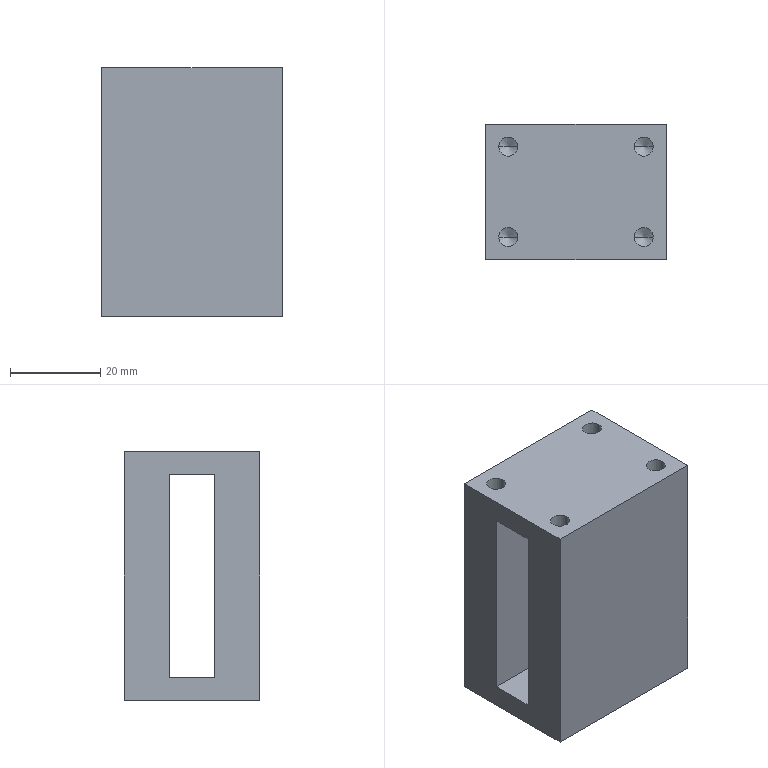Component | SolidWorks | 01-14MarkingMachineMountingSeatPlate-1 | 1 solid | 28 faces | box 40 x 30 x 55 mm | volume 46926 mm3 | cylinder 10 | plane 10 | cone 8 | commonest cylinder face diameters 4.2 x8 6.8 x2 | material A3 Steel
build123d program:
from build123d import *

# Parameters (mm, degrees)
SKETCH1_W             = 55
SKETCH1_H             = 30
SKETCH1_W_2           = 45
SKETCH1_H_2           = 10
BOSS_EXTRUDE1_DEPTH   = 20
M8_TAPPED_HOLE1_D     = 6.8
M8_TAPPED_HOLE1_DEPTH = 10
M5_TAPPED_HOLE1_D     = 4.2
M5_TAPPED_HOLE1_DEPTH = 12.4
M5_TAPPED_HOLE1_TIP   = 1.262


with BuildPart() as part:
    # Sketch1 → Boss-Extrude1 (new, symmetric)
    with BuildSketch(Plane.XY):
        Rectangle(SKETCH1_W, SKETCH1_H)
        Rectangle(SKETCH1_W_2, SKETCH1_H_2, mode=Mode.SUBTRACT)
    extrude(amount=BOSS_EXTRUDE1_DEPTH, both=True)

    # M8 Tapped Hole1
    with Locations(Plane.ZX.offset(15)):
        with Locations((0, 0)):
            Hole(M8_TAPPED_HOLE1_D / 2, depth=M8_TAPPED_HOLE1_DEPTH)

    # M5 Tapped Hole1
    with Locations(Plane(origin=(-27.5, 10, -15), x_dir=(0, 0, -1), z_dir=(-1, 0, 0))):
        with Locations((0, 0), (0, 20), (-30, 0), (-30, 20)):
            Hole(M5_TAPPED_HOLE1_D / 2, depth=M5_TAPPED_HOLE1_DEPTH)
            with Locations((0, 0, -(M5_TAPPED_HOLE1_DEPTH + M5_TAPPED_HOLE1_TIP / 2))):  # 118° drill point
                Cone(0, M5_TAPPED_HOLE1_D / 2, M5_TAPPED_HOLE1_TIP, mode=Mode.SUBTRACT)


solid = part.part

# Placed as in the assembly
solid = solid.moved(Location((-179.532, 2.41, -167.5), (0, 90, 0)))
STEP:
#1=CARTESIAN_POINT('',(-7.741,0.4886,-6.));
#2=VERTEX_POINT('',#1);
#3=CARTESIAN_POINT('',(-7.576,0.4886,-6.));
#4=VERTEX_POINT('',#3);
#5=CARTESIAN_POINT('',(-7.659,0.4886,-6.));
#6=DIRECTION('',(0.,-0.,1.));
#7=DIRECTION('',(1.,0.,0.));
#8=AXIS2_PLACEMENT_3D('',#5,#6,#7);
#9=CIRCLE('',#8,0.08268);
#10=EDGE_CURVE('',#2,#4,#9,.T.);
#11=ORIENTED_EDGE('',*,*,#10,.F.);
#12=CARTESIAN_POINT('',(-7.741,0.4886,-5.512));
#13=VERTEX_POINT('',#12);
#14=CARTESIAN_POINT('',(-7.741,0.4886,-5.512));
#15=DIRECTION('',(0.,-0.,1.));
#16=VECTOR('',#15,39.37);
#17=LINE('',#14,#16);
#18=EDGE_CURVE('',#2,#13,#17,.T.);
#19=ORIENTED_EDGE('',*,*,#18,.T.);
#20=CARTESIAN_POINT('',(-7.576,0.4886,-5.512));
#21=VERTEX_POINT('',#20);
#22=CARTESIAN_POINT('',(-7.659,0.4886,-5.512));
#23=DIRECTION('',(0.,-0.,1.));
#24=DIRECTION('',(1.,0.,0.));
#25=AXIS2_PLACEMENT_3D('',#22,#23,#24);
#26=CIRCLE('',#25,0.08268);
#27=EDGE_CURVE('',#13,#21,#26,.T.);
#28=ORIENTED_EDGE('',*,*,#27,.T.);
#29=CARTESIAN_POINT('',(-7.576,0.4886,-5.512));
#30=DIRECTION('',(0.,-0.,1.));
#31=VECTOR('',#30,39.37);
#32=LINE('',#29,#31);
#33=EDGE_CURVE('',#4,#21,#32,.T.);
#34=ORIENTED_EDGE('',*,*,#33,.F.);
#35=EDGE_LOOP('',(#11,#19,#28,#34));
#36=FACE_OUTER_BOUND('',#35,.T.);
#37=CARTESIAN_POINT('',(-7.659,0.4886,-5.512));
#38=DIRECTION('',(0.,-0.,1.));
#39=DIRECTION('',(1.,0.,0.));
#40=AXIS2_PLACEMENT_3D('',#37,#38,#39);
#41=CYLINDRICAL_SURFACE('',#40,0.08268);
#42=ADVANCED_FACE('',(#36),#41,.F.);
#43=CARTESIAN_POINT('',(-7.659,0.4886,-6.05));
#44=VERTEX_POINT('',#43);
#45=CARTESIAN_POINT('',(-7.576,0.4886,-6.));
#46=DIRECTION('',(0.8572,0.,0.515));
#47=VECTOR('',#46,39.37);
#48=LINE('',#45,#47);
#49=EDGE_CURVE('',#44,#4,#48,.T.);
#50=ORIENTED_EDGE('',*,*,#49,.F.);
#51=CARTESIAN_POINT('',(-7.741,0.4886,-6.));
#52=DIRECTION('',(-0.8572,-0.,0.515));
#53=VECTOR('',#52,39.37);
#54=LINE('',#51,#53);
#55=EDGE_CURVE('',#44,#2,#54,.T.);
#56=ORIENTED_EDGE('',*,*,#55,.T.);
#57=ORIENTED_EDGE('',*,*,#10,.T.);
#58=EDGE_LOOP('',(#50,#56,#57));
#59=FACE_OUTER_BOUND('',#58,.T.);
#60=CARTESIAN_POINT('',(-7.659,0.4886,-6.));
#61=DIRECTION('',(0.,-0.,1.));
#62=DIRECTION('',(1.,0.,0.));
#63=AXIS2_PLACEMENT_3D('',#60,#61,#62);
#64=CONICAL_SURFACE('',#63,0.08268,1.03);
#65=ADVANCED_FACE('',(#59),#64,.F.);
#66=CARTESIAN_POINT('',(-7.741,-0.2988,-6.));
#67=VERTEX_POINT('',#66);
#68=CARTESIAN_POINT('',(-7.576,-0.2988,-6.));
#69=VERTEX_POINT('',#68);
#70=CARTESIAN_POINT('',(-7.659,-0.2988,-6.));
#71=DIRECTION('',(0.,-0.,1.));
#72=DIRECTION('',(1.,0.,0.));
#73=AXIS2_PLACEMENT_3D('',#70,#71,#72);
#74=CIRCLE('',#73,0.08268);
#75=EDGE_CURVE('',#67,#69,#74,.T.);
#76=ORIENTED_EDGE('',*,*,#75,.F.);
#77=CARTESIAN_POINT('',(-7.741,-0.2988,-5.512));
#78=VERTEX_POINT('',#77);
#79=CARTESIAN_POINT('',(-7.741,-0.2988,-5.512));
#80=DIRECTION('',(0.,-0.,1.));
#81=VECTOR('',#80,39.37);
#82=LINE('',#79,#81);
#83=EDGE_CURVE('',#67,#78,#82,.T.);
#84=ORIENTED_EDGE('',*,*,#83,.T.);
#85=CARTESIAN_POINT('',(-7.576,-0.2988,-5.512));
#86=VERTEX_POINT('',#85);
#87=CARTESIAN_POINT('',(-7.659,-0.2988,-5.512));
#88=DIRECTION('',(0.,-0.,1.));
#89=DIRECTION('',(1.,0.,0.));
#90=AXIS2_PLACEMENT_3D('',#87,#88,#89);
#91=CIRCLE('',#90,0.08268);
#92=EDGE_CURVE('',#78,#86,#91,.T.);
#93=ORIENTED_EDGE('',*,*,#92,.T.);
#94=CARTESIAN_POINT('',(-7.576,-0.2988,-5.512));
#95=DIRECTION('',(0.,-0.,1.));
#96=VECTOR('',#95,39.37);
#97=LINE('',#94,#96);
#98=EDGE_CURVE('',#69,#86,#97,.T.);
#99=ORIENTED_EDGE('',*,*,#98,.F.);
#100=EDGE_LOOP('',(#76,#84,#93,#99));
#101=FACE_OUTER_BOUND('',#100,.T.);
#102=CARTESIAN_POINT('',(-7.659,-0.2988,-5.512));
#103=DIRECTION('',(0.,-0.,1.));
#104=DIRECTION('',(1.,0.,0.));
#105=AXIS2_PLACEMENT_3D('',#102,#103,#104);
#106=CYLINDRICAL_SURFACE('',#105,0.08268);
#107=ADVANCED_FACE('',(#101),#106,.F.);
#108=CARTESIAN_POINT('',(-7.659,-0.2988,-6.05));
#109=VERTEX_POINT('',#108);
#110=CARTESIAN_POINT('',(-7.576,-0.2988,-6.));
#111=DIRECTION('',(0.8572,0.,0.515));
#112=VECTOR('',#111,39.37);
#113=LINE('',#110,#112);
#114=EDGE_CURVE('',#109,#69,#113,.T.);
#115=ORIENTED_EDGE('',*,*,#114,.F.);
#116=CARTESIAN_POINT('',(-7.741,-0.2988,-6.));
#117=DIRECTION('',(-0.8572,-0.,0.515));
#118=VECTOR('',#117,39.37);
#119=LINE('',#116,#118);
#120=EDGE_CURVE('',#109,#67,#119,.T.);
#121=ORIENTED_EDGE('',*,*,#120,.T.);
#122=ORIENTED_EDGE('',*,*,#75,.T.);
#123=EDGE_LOOP('',(#115,#121,#122));
#124=FACE_OUTER_BOUND('',#123,.T.);
#125=CARTESIAN_POINT('',(-7.659,-0.2988,-6.));
#126=DIRECTION('',(0.,-0.,1.));
#127=DIRECTION('',(1.,0.,0.));
#128=AXIS2_PLACEMENT_3D('',#125,#126,#127);
#129=CONICAL_SURFACE('',#128,0.08268,1.03);
#130=ADVANCED_FACE('',(#124),#129,.F.);
#131=CARTESIAN_POINT('',(-6.56,0.4886,-6.));
#132=VERTEX_POINT('',#131);
#133=CARTESIAN_POINT('',(-6.395,0.4886,-6.));
#134=VERTEX_POINT('',#133);
#135=CARTESIAN_POINT('',(-6.478,0.4886,-6.));
#136=DIRECTION('',(0.,-0.,1.));
#137=DIRECTION('',(1.,0.,0.));
#138=AXIS2_PLACEMENT_3D('',#135,#136,#137);
#139=CIRCLE('',#138,0.08268);
#140=EDGE_CURVE('',#132,#134,#139,.T.);
#141=ORIENTED_EDGE('',*,*,#140,.F.);
#142=CARTESIAN_POINT('',(-6.56,0.4886,-5.512));
#143=VERTEX_POINT('',#142);
#144=CARTESIAN_POINT('',(-6.56,0.4886,-5.512));
#145=DIRECTION('',(0.,-0.,1.));
#146=VECTOR('',#145,39.37);
#147=LINE('',#144,#146);
#148=EDGE_CURVE('',#132,#143,#147,.T.);
#149=ORIENTED_EDGE('',*,*,#148,.T.);
#150=CARTESIAN_POINT('',(-6.395,0.4886,-5.512));
#151=VERTEX_POINT('',#150);
#152=CARTESIAN_POINT('',(-6.478,0.4886,-5.512));
#153=DIRECTION('',(0.,-0.,1.));
#154=DIRECTION('',(1.,0.,0.));
#155=AXIS2_PLACEMENT_3D('',#152,#153,#154);
#156=CIRCLE('',#155,0.08268);
#157=EDGE_CURVE('',#143,#151,#156,.T.);
#158=ORIENTED_EDGE('',*,*,#157,.T.);
#159=CARTESIAN_POINT('',(-6.395,0.4886,-5.512));
#160=DIRECTION('',(0.,-0.,1.));
#161=VECTOR('',#160,39.37);
#162=LINE('',#159,#161);
#163=EDGE_CURVE('',#134,#151,#162,.T.);
#164=ORIENTED_EDGE('',*,*,#163,.F.);
#165=EDGE_LOOP('',(#141,#149,#158,#164));
#166=FACE_OUTER_BOUND('',#165,.T.);
#167=CARTESIAN_POINT('',(-6.478,0.4886,-5.512));
#168=DIRECTION('',(0.,-0.,1.));
#169=DIRECTION('',(1.,0.,0.));
#170=AXIS2_PLACEMENT_3D('',#167,#168,#169);
#171=CYLINDRICAL_SURFACE('',#170,0.08268);
#172=ADVANCED_FACE('',(#166),#171,.F.);
#173=CARTESIAN_POINT('',(-6.478,0.4886,-6.05));
#174=VERTEX_POINT('',#173);
#175=CARTESIAN_POINT('',(-6.395,0.4886,-6.));
#176=DIRECTION('',(0.8572,0.,0.515));
#177=VECTOR('',#176,39.37);
#178=LINE('',#175,#177);
#179=EDGE_CURVE('',#174,#134,#178,.T.);
#180=ORIENTED_EDGE('',*,*,#179,.F.);
#181=CARTESIAN_POINT('',(-6.56,0.4886,-6.));
#182=DIRECTION('',(-0.8572,-0.,0.515));
#183=VECTOR('',#182,39.37);
#184=LINE('',#181,#183);
#185=EDGE_CURVE('',#174,#132,#184,.T.);
#186=ORIENTED_EDGE('',*,*,#185,.T.);
#187=ORIENTED_EDGE('',*,*,#140,.T.);
#188=EDGE_LOOP('',(#180,#186,#187));
#189=FACE_OUTER_BOUND('',#188,.T.);
#190=CARTESIAN_POINT('',(-6.478,0.4886,-6.));
#191=DIRECTION('',(0.,-0.,1.));
#192=DIRECTION('',(1.,0.,0.));
#193=AXIS2_PLACEMENT_3D('',#190,#191,#192);
#194=CONICAL_SURFACE('',#193,0.08268,1.03);
#195=ADVANCED_FACE('',(#189),#194,.F.);
#196=CARTESIAN_POINT('',(-6.56,-0.2988,-6.));
#197=VERTEX_POINT('',#196);
#198=CARTESIAN_POINT('',(-6.395,-0.2988,-6.));
#199=VERTEX_POINT('',#198);
#200=CARTESIAN_POINT('',(-6.478,-0.2988,-6.));
#201=DIRECTION('',(0.,-0.,1.));
#202=DIRECTION('',(1.,0.,0.));
#203=AXIS2_PLACEMENT_3D('',#200,#201,#202);
#204=CIRCLE('',#203,0.08268);
#205=EDGE_CURVE('',#197,#199,#204,.T.);
#206=ORIENTED_EDGE('',*,*,#205,.F.);
#207=CARTESIAN_POINT('',(-6.56,-0.2988,-5.512));
#208=VERTEX_POINT('',#207);
#209=CARTESIAN_POINT('',(-6.56,-0.2988,-5.512));
#210=DIRECTION('',(0.,-0.,1.));
#211=VECTOR('',#210,39.37);
#212=LINE('',#209,#211);
#213=EDGE_CURVE('',#197,#208,#212,.T.);
#214=ORIENTED_EDGE('',*,*,#213,.T.);
#215=CARTESIAN_POINT('',(-6.395,-0.2988,-5.512));
#216=VERTEX_POINT('',#215);
#217=CARTESIAN_POINT('',(-6.478,-0.2988,-5.512));
#218=DIRECTION('',(0.,-0.,1.));
#219=DIRECTION('',(1.,0.,0.));
#220=AXIS2_PLACEMENT_3D('',#217,#218,#219);
#221=CIRCLE('',#220,0.08268);
#222=EDGE_CURVE('',#208,#216,#221,.T.);
#223=ORIENTED_EDGE('',*,*,#222,.T.);
#224=CARTESIAN_POINT('',(-6.395,-0.2988,-5.512));
#225=DIRECTION('',(0.,-0.,1.));
#226=VECTOR('',#225,39.37);
#227=LINE('',#224,#226);
#228=EDGE_CURVE('',#199,#216,#227,.T.);
#229=ORIENTED_EDGE('',*,*,#228,.F.);
#230=EDGE_LOOP('',(#206,#214,#223,#229));
#231=FACE_OUTER_BOUND('',#230,.T.);
#232=CARTESIAN_POINT('',(-6.478,-0.2988,-5.512));
#233=DIRECTION('',(0.,-0.,1.));
#234=DIRECTION('',(1.,0.,0.));
#235=AXIS2_PLACEMENT_3D('',#232,#233,#234);
#236=CYLINDRICAL_SURFACE('',#235,0.08268);
#237=ADVANCED_FACE('',(#231),#236,.F.);
#238=CARTESIAN_POINT('',(-6.478,-0.2988,-6.05));
#239=VERTEX_POINT('',#238);
#240=CARTESIAN_POINT('',(-6.395,-0.2988,-6.));
#241=DIRECTION('',(0.8572,0.,0.515));
#242=VECTOR('',#241,39.37);
#243=LINE('',#240,#242);
#244=EDGE_CURVE('',#239,#199,#243,.T.);
#245=ORIENTED_EDGE('',*,*,#244,.F.);
#246=CARTESIAN_POINT('',(-6.56,-0.2988,-6.));
#247=DIRECTION('',(-0.8572,-0.,0.515));
#248=VECTOR('',#247,39.37);
#249=LINE('',#246,#248);
#250=EDGE_CURVE('',#239,#197,#249,.T.);
#251=ORIENTED_EDGE('',*,*,#250,.T.);
#252=ORIENTED_EDGE('',*,*,#205,.T.);
#253=EDGE_LOOP('',(#245,#251,#252));
#254=FACE_OUTER_BOUND('',#253,.T.);
#255=CARTESIAN_POINT('',(-6.478,-0.2988,-6.));
#256=DIRECTION('',(0.,-0.,1.));
#257=DIRECTION('',(1.,0.,0.));
#258=AXIS2_PLACEMENT_3D('',#255,#256,#257);
#259=CONICAL_SURFACE('',#258,0.08268,1.03);
#260=ADVANCED_FACE('',(#254),#259,.F.);
#261=CARTESIAN_POINT('',(-6.934,0.2918,-6.594));
#262=VERTEX_POINT('',#261);
#263=CARTESIAN_POINT('',(-7.202,0.2918,-6.594));
#264=VERTEX_POINT('',#263);
#265=CARTESIAN_POINT('',(-7.068,0.2918,-6.594));
#266=DIRECTION('',(0.,-1.,-0.));
#267=DIRECTION('',(-1.,0.,0.));
#268=AXIS2_PLACEMENT_3D('',#265,#266,#267);
#269=CIRCLE('',#268,0.1339);
#270=EDGE_CURVE('',#262,#264,#269,.T.);
#271=ORIENTED_EDGE('',*,*,#270,.T.);
#272=CARTESIAN_POINT('',(-7.202,0.6855,-6.594));
#273=VERTEX_POINT('',#272);
#274=CARTESIAN_POINT('',(-7.202,0.6855,-6.594));
#275=DIRECTION('',(-0.,1.,0.));
#276=VECTOR('',#275,39.37);
#277=LINE('',#274,#276);
#278=EDGE_CURVE('',#264,#273,#277,.T.);
#279=ORIENTED_EDGE('',*,*,#278,.T.);
#280=CARTESIAN_POINT('',(-6.934,0.6855,-6.594));
#281=VERTEX_POINT('',#280);
#282=CARTESIAN_POINT('',(-7.068,0.6855,-6.594));
#283=DIRECTION('',(-0.,1.,0.));
#284=DIRECTION('',(1.,0.,0.));
#285=AXIS2_PLACEMENT_3D('',#282,#283,#284);
#286=CIRCLE('',#285,0.1339);
#287=EDGE_CURVE('',#273,#281,#286,.T.);
#288=ORIENTED_EDGE('',*,*,#287,.T.);
#289=CARTESIAN_POINT('',(-6.934,0.6855,-6.594));
#290=DIRECTION('',(-0.,1.,0.));
#291=VECTOR('',#290,39.37);
#292=LINE('',#289,#291);
#293=EDGE_CURVE('',#262,#281,#292,.T.);
#294=ORIENTED_EDGE('',*,*,#293,.F.);
#295=EDGE_LOOP('',(#271,#279,#288,#294));
#296=FACE_OUTER_BOUND('',#295,.T.);
#297=CARTESIAN_POINT('',(-7.068,0.6855,-6.594));
#298=DIRECTION('',(-0.,1.,0.));
#299=DIRECTION('',(1.,0.,0.));
#300=AXIS2_PLACEMENT_3D('',#297,#298,#299);
#301=CYLINDRICAL_SURFACE('',#300,0.1339);
#302=ADVANCED_FACE('',(#296),#301,.F.);
#303=CARTESIAN_POINT('',(-6.281,-0.4957,-7.677));
#304=VERTEX_POINT('',#303);
#305=CARTESIAN_POINT('',(-6.281,0.6855,-7.677));
#306=VERTEX_POINT('',#305);
#307=CARTESIAN_POINT('',(-6.281,-0.4957,-7.677));
#308=DIRECTION('',(-0.,1.,0.));
#309=VECTOR('',#308,39.37);
#310=LINE('',#307,#309);
#311=EDGE_CURVE('',#304,#306,#310,.T.);
#312=ORIENTED_EDGE('',*,*,#311,.T.);
#313=CARTESIAN_POINT('',(-6.281,0.6855,-5.512));
#314=VERTEX_POINT('',#313);
#315=CARTESIAN_POINT('',(-6.281,0.6855,-5.512));
#316=DIRECTION('',(0.,-0.,1.));
#317=VECTOR('',#316,39.37);
#318=LINE('',#315,#317);
#319=EDGE_CURVE('',#306,#314,#318,.T.);
#320=ORIENTED_EDGE('',*,*,#319,.T.);
#321=CARTESIAN_POINT('',(-6.281,-0.4957,-5.512));
#322=VERTEX_POINT('',#321);
#323=CARTESIAN_POINT('',(-6.281,-0.4957,-5.512));
#324=DIRECTION('',(0.,-1.,-0.));
#325=VECTOR('',#324,39.37);
#326=LINE('',#323,#325);
#327=EDGE_CURVE('',#314,#322,#326,.T.);
#328=ORIENTED_EDGE('',*,*,#327,.T.);
#329=CARTESIAN_POINT('',(-6.281,-0.4957,-5.512));
#330=DIRECTION('',(-0.,0.,-1.));
#331=VECTOR('',#330,39.37);
#332=LINE('',#329,#331);
#333=EDGE_CURVE('',#322,#304,#332,.T.);
#334=ORIENTED_EDGE('',*,*,#333,.T.);
#335=EDGE_LOOP('',(#312,#320,#328,#334));
#336=FACE_OUTER_BOUND('',#335,.T.);
#337=CARTESIAN_POINT('',(-6.281,-0.102,-7.48));
#338=VERTEX_POINT('',#337);
#339=CARTESIAN_POINT('',(-6.281,0.2918,-7.48));
#340=VERTEX_POINT('',#339);
#341=CARTESIAN_POINT('',(-6.281,-0.102,-7.48));
#342=DIRECTION('',(-0.,1.,0.));
#343=VECTOR('',#342,39.37);
#344=LINE('',#341,#343);
#345=EDGE_CURVE('',#338,#340,#344,.T.);
#346=ORIENTED_EDGE('',*,*,#345,.F.);
#347=CARTESIAN_POINT('',(-6.281,-0.102,-5.709));
#348=VERTEX_POINT('',#347);
#349=CARTESIAN_POINT('',(-6.281,-0.102,-5.709));
#350=DIRECTION('',(-0.,0.,-1.));
#351=VECTOR('',#350,39.37);
#352=LINE('',#349,#351);
#353=EDGE_CURVE('',#348,#338,#352,.T.);
#354=ORIENTED_EDGE('',*,*,#353,.F.);
#355=CARTESIAN_POINT('',(-6.281,0.2918,-5.709));
#356=VERTEX_POINT('',#355);
#357=CARTESIAN_POINT('',(-6.281,-0.102,-5.709));
#358=DIRECTION('',(0.,-1.,-0.));
#359=VECTOR('',#358,39.37);
#360=LINE('',#357,#359);
#361=EDGE_CURVE('',#356,#348,#360,.T.);
#362=ORIENTED_EDGE('',*,*,#361,.F.);
#363=CARTESIAN_POINT('',(-6.281,0.2918,-5.709));
#364=DIRECTION('',(0.,-0.,1.));
#365=VECTOR('',#364,39.37);
#366=LINE('',#363,#365);
#367=EDGE_CURVE('',#340,#356,#366,.T.);
#368=ORIENTED_EDGE('',*,*,#367,.F.);
#369=EDGE_LOOP('',(#346,#354,#362,#368));
#370=FACE_BOUND('',#369,.T.);
#371=CARTESIAN_POINT('',(-6.281,0.0949,-6.594));
#372=DIRECTION('',(-1.,-0.,0.));
#373=DIRECTION('',(0.,-0.,1.));
#374=AXIS2_PLACEMENT_3D('',#371,#372,#373);
#375=PLANE('',#374);
#376=ADVANCED_FACE('',(#336,#370),#375,.F.);
#377=CARTESIAN_POINT('',(-7.856,-0.4957,-7.677));
#378=VERTEX_POINT('',#377);
#379=CARTESIAN_POINT('',(-7.856,0.6855,-7.677));
#380=VERTEX_POINT('',#379);
#381=CARTESIAN_POINT('',(-7.856,-0.4957,-7.677));
#382=DIRECTION('',(-0.,1.,0.));
#383=VECTOR('',#382,39.37);
#384=LINE('',#381,#383);
#385=EDGE_CURVE('',#378,#380,#384,.T.);
#386=ORIENTED_EDGE('',*,*,#385,.F.);
#387=CARTESIAN_POINT('',(-7.856,-0.4957,-5.512));
#388=VERTEX_POINT('',#387);
#389=CARTESIAN_POINT('',(-7.856,-0.4957,-5.512));
#390=DIRECTION('',(-0.,0.,-1.));
#391=VECTOR('',#390,39.37);
#392=LINE('',#389,#391);
#393=EDGE_CURVE('',#388,#378,#392,.T.);
#394=ORIENTED_EDGE('',*,*,#393,.F.);
#395=CARTESIAN_POINT('',(-7.856,0.6855,-5.512));
#396=VERTEX_POINT('',#395);
#397=CARTESIAN_POINT('',(-7.856,-0.4957,-5.512));
#398=DIRECTION('',(0.,-1.,-0.));
#399=VECTOR('',#398,39.37);
#400=LINE('',#397,#399);
#401=EDGE_CURVE('',#396,#388,#400,.T.);
#402=ORIENTED_EDGE('',*,*,#401,.F.);
#403=CARTESIAN_POINT('',(-7.856,0.6855,-5.512));
#404=DIRECTION('',(0.,-0.,1.));
#405=VECTOR('',#404,39.37);
#406=LINE('',#403,#405);
#407=EDGE_CURVE('',#380,#396,#406,.T.);
#408=ORIENTED_EDGE('',*,*,#407,.F.);
#409=EDGE_LOOP('',(#386,#394,#402,#408));
#410=FACE_OUTER_BOUND('',#409,.T.);
#411=CARTESIAN_POINT('',(-7.856,-0.102,-5.709));
#412=VERTEX_POINT('',#411);
#413=CARTESIAN_POINT('',(-7.856,-0.102,-7.48));
#414=VERTEX_POINT('',#413);
#415=CARTESIAN_POINT('',(-7.856,-0.102,-5.709));
#416=DIRECTION('',(-0.,0.,-1.));
#417=VECTOR('',#416,39.37);
#418=LINE('',#415,#417);
#419=EDGE_CURVE('',#412,#414,#418,.T.);
#420=ORIENTED_EDGE('',*,*,#419,.T.);
#421=CARTESIAN_POINT('',(-7.856,0.2918,-7.48));
#422=VERTEX_POINT('',#421);
#423=CARTESIAN_POINT('',(-7.856,-0.102,-7.48));
#424=DIRECTION('',(-0.,1.,0.));
#425=VECTOR('',#424,39.37);
#426=LINE('',#423,#425);
#427=EDGE_CURVE('',#414,#422,#426,.T.);
#428=ORIENTED_EDGE('',*,*,#427,.T.);
#429=CARTESIAN_POINT('',(-7.856,0.2918,-5.709));
#430=VERTEX_POINT('',#429);
#431=CARTESIAN_POINT('',(-7.856,0.2918,-5.709));
#432=DIRECTION('',(0.,-0.,1.));
#433=VECTOR('',#432,39.37);
#434=LINE('',#431,#433);
#435=EDGE_CURVE('',#422,#430,#434,.T.);
#436=ORIENTED_EDGE('',*,*,#435,.T.);
#437=CARTESIAN_POINT('',(-7.856,-0.102,-5.709));
#438=DIRECTION('',(0.,-1.,-0.));
#439=VECTOR('',#438,39.37);
#440=LINE('',#437,#439);
#441=EDGE_CURVE('',#430,#412,#440,.T.);
#442=ORIENTED_EDGE('',*,*,#441,.T.);
#443=EDGE_LOOP('',(#420,#428,#436,#442));
#444=FACE_BOUND('',#443,.T.);
#445=CARTESIAN_POINT('',(-7.856,0.0949,-6.594));
#446=DIRECTION('',(-1.,-0.,0.));
#447=DIRECTION('',(0.,-0.,1.));
#448=AXIS2_PLACEMENT_3D('',#445,#446,#447);
#449=PLANE('',#448);
#450=ADVANCED_FACE('',(#410,#444),#449,.T.);
#451=ORIENTED_EDGE('',*,*,#385,.T.);
#452=CARTESIAN_POINT('',(-6.281,0.6855,-7.677));
#453=DIRECTION('',(-1.,-0.,0.));
#454=VECTOR('',#453,39.37);
#455=LINE('',#452,#454);
#456=EDGE_CURVE('',#306,#380,#455,.T.);
#457=ORIENTED_EDGE('',*,*,#456,.F.);
#458=ORIENTED_EDGE('',*,*,#311,.F.);
#459=CARTESIAN_POINT('',(-6.281,-0.4957,-7.677));
#460=DIRECTION('',(-1.,-0.,0.));
#461=VECTOR('',#460,39.37);
#462=LINE('',#459,#461);
#463=EDGE_CURVE('',#304,#378,#462,.T.);
#464=ORIENTED_EDGE('',*,*,#463,.T.);
#465=EDGE_LOOP('',(#451,#457,#458,#464));
#466=FACE_OUTER_BOUND('',#465,.T.);
#467=CARTESIAN_POINT('',(-6.281,-0.4957,-7.677));
#468=DIRECTION('',(0.,-0.,1.));
#469=DIRECTION('',(1.,0.,-0.));
#470=AXIS2_PLACEMENT_3D('',#467,#468,#469);
#471=PLANE('',#470);
#472=ADVANCED_FACE('',(#466),#471,.F.);
#473=CARTESIAN_POINT('',(-7.068,0.6855,-6.594));
#474=DIRECTION('',(-0.,1.,0.));
#475=DIRECTION('',(1.,0.,0.));
#476=AXIS2_PLACEMENT_3D('',#473,#474,#475);
#477=CIRCLE('',#476,0.1339);
#478=EDGE_CURVE('',#281,#273,#477,.T.);
#479=ORIENTED_EDGE('',*,*,#478,.F.);
#480=ORIENTED_EDGE('',*,*,#287,.F.);
#481=EDGE_LOOP('',(#479,#480));
#482=FACE_BOUND('',#481,.T.);
#483=ORIENTED_EDGE('',*,*,#407,.T.);
#484=CARTESIAN_POINT('',(-6.281,0.6855,-5.512));
#485=DIRECTION('',(-1.,-0.,0.));
#486=VECTOR('',#485,39.37);
#487=LINE('',#484,#486);
#488=EDGE_CURVE('',#314,#396,#487,.T.);
#489=ORIENTED_EDGE('',*,*,#488,.F.);
#490=ORIENTED_EDGE('',*,*,#319,.F.);
#491=ORIENTED_EDGE('',*,*,#456,.T.);
#492=EDGE_LOOP('',(#483,#489,#490,#491));
#493=FACE_OUTER_BOUND('',#492,.T.);
#494=CARTESIAN_POINT('',(-6.281,0.6855,-5.512));
#495=DIRECTION('',(0.,-1.,-0.));
#496=DIRECTION('',(-1.,-0.,0.));
#497=AXIS2_PLACEMENT_3D('',#494,#495,#496);
#498=PLANE('',#497);
#499=ADVANCED_FACE('',(#482,#493),#498,.F.);
#500=CARTESIAN_POINT('',(-7.659,0.4886,-5.512));
#501=DIRECTION('',(0.,-0.,1.));
#502=DIRECTION('',(1.,0.,0.));
#503=AXIS2_PLACEMENT_3D('',#500,#501,#502);
#504=CIRCLE('',#503,0.08268);
#505=EDGE_CURVE('',#21,#13,#504,.T.);
#506=ORIENTED_EDGE('',*,*,#505,.F.);
#507=ORIENTED_EDGE('',*,*,#27,.F.);
#508=EDGE_LOOP('',(#506,#507));
#509=FACE_BOUND('',#508,.T.);
#510=CARTESIAN_POINT('',(-7.659,-0.2988,-5.512));
#511=DIRECTION('',(0.,-0.,1.));
#512=DIRECTION('',(1.,0.,0.));
#513=AXIS2_PLACEMENT_3D('',#510,#511,#512);
#514=CIRCLE('',#513,0.08268);
#515=EDGE_CURVE('',#86,#78,#514,.T.);
#516=ORIENTED_EDGE('',*,*,#515,.F.);
#517=ORIENTED_EDGE('',*,*,#92,.F.);
#518=EDGE_LOOP('',(#516,#517));
#519=FACE_BOUND('',#518,.T.);
#520=CARTESIAN_POINT('',(-6.478,0.4886,-5.512));
#521=DIRECTION('',(0.,-0.,1.));
#522=DIRECTION('',(1.,0.,0.));
#523=AXIS2_PLACEMENT_3D('',#520,#521,#522);
#524=CIRCLE('',#523,0.08268);
#525=EDGE_CURVE('',#151,#143,#524,.T.);
#526=ORIENTED_EDGE('',*,*,#525,.F.);
#527=ORIENTED_EDGE('',*,*,#157,.F.);
#528=EDGE_LOOP('',(#526,#527));
#529=FACE_BOUND('',#528,.T.);
#530=CARTESIAN_POINT('',(-6.478,-0.2988,-5.512));
#531=DIRECTION('',(0.,-0.,1.));
#532=DIRECTION('',(1.,0.,0.));
#533=AXIS2_PLACEMENT_3D('',#530,#531,#532);
#534=CIRCLE('',#533,0.08268);
#535=EDGE_CURVE('',#216,#208,#534,.T.);
#536=ORIENTED_EDGE('',*,*,#535,.F.);
#537=ORIENTED_EDGE('',*,*,#222,.F.);
#538=EDGE_LOOP('',(#536,#537));
#539=FACE_BOUND('',#538,.T.);
#540=ORIENTED_EDGE('',*,*,#401,.T.);
#541=CARTESIAN_POINT('',(-6.281,-0.4957,-5.512));
#542=DIRECTION('',(-1.,-0.,0.));
#543=VECTOR('',#542,39.37);
#544=LINE('',#541,#543);
#545=EDGE_CURVE('',#322,#388,#544,.T.);
#546=ORIENTED_EDGE('',*,*,#545,.F.);
#547=ORIENTED_EDGE('',*,*,#327,.F.);
#548=ORIENTED_EDGE('',*,*,#488,.T.);
#549=EDGE_LOOP('',(#540,#546,#547,#548));
#550=FACE_OUTER_BOUND('',#549,.T.);
#551=CARTESIAN_POINT('',(-6.281,-0.4957,-5.512));
#552=DIRECTION('',(-0.,0.,-1.));
#553=DIRECTION('',(-1.,-0.,0.));
#554=AXIS2_PLACEMENT_3D('',#551,#552,#553);
#555=PLANE('',#554);
#556=ADVANCED_FACE('',(#509,#519,#529,#539,#550),#555,.F.);
#557=ORIENTED_EDGE('',*,*,#393,.T.);
#558=ORIENTED_EDGE('',*,*,#463,.F.);
#559=ORIENTED_EDGE('',*,*,#333,.F.);
#560=ORIENTED_EDGE('',*,*,#545,.T.);
#561=EDGE_LOOP('',(#557,#558,#559,#560));
#562=FACE_OUTER_BOUND('',#561,.T.);
#563=CARTESIAN_POINT('',(-6.281,-0.4957,-5.512));
#564=DIRECTION('',(-0.,1.,0.));
#565=DIRECTION('',(1.,0.,-0.));
#566=AXIS2_PLACEMENT_3D('',#563,#564,#565);
#567=PLANE('',#566);
#568=ADVANCED_FACE('',(#562),#567,.F.);
#569=ORIENTED_EDGE('',*,*,#427,.F.);
#570=CARTESIAN_POINT('',(-6.281,-0.102,-7.48));
#571=DIRECTION('',(-1.,-0.,0.));
#572=VECTOR('',#571,39.37);
#573=LINE('',#570,#572);
#574=EDGE_CURVE('',#338,#414,#573,.T.);
#575=ORIENTED_EDGE('',*,*,#574,.F.);
#576=ORIENTED_EDGE('',*,*,#345,.T.);
#577=CARTESIAN_POINT('',(-6.281,0.2918,-7.48));
#578=DIRECTION('',(-1.,-0.,0.));
#579=VECTOR('',#578,39.37);
#580=LINE('',#577,#579);
#581=EDGE_CURVE('',#340,#422,#580,.T.);
#582=ORIENTED_EDGE('',*,*,#581,.T.);
#583=EDGE_LOOP('',(#569,#575,#576,#582));
#584=FACE_OUTER_BOUND('',#583,.T.);
#585=CARTESIAN_POINT('',(-6.281,-0.102,-7.48));
#586=DIRECTION('',(0.,-0.,1.));
#587=DIRECTION('',(1.,0.,-0.));
#588=AXIS2_PLACEMENT_3D('',#585,#586,#587);
#589=PLANE('',#588);
#590=ADVANCED_FACE('',(#584),#589,.T.);
#591=ORIENTED_EDGE('',*,*,#270,.F.);
#592=CARTESIAN_POINT('',(-7.068,0.2918,-6.594));
#593=DIRECTION('',(0.,-1.,-0.));
#594=DIRECTION('',(-1.,0.,0.));
#595=AXIS2_PLACEMENT_3D('',#592,#593,#594);
#596=CIRCLE('',#595,0.1339);
#597=EDGE_CURVE('',#264,#262,#596,.T.);
#598=ORIENTED_EDGE('',*,*,#597,.F.);
#599=EDGE_LOOP('',(#591,#598));
#600=FACE_BOUND('',#599,.T.);
#601=ORIENTED_EDGE('',*,*,#435,.F.);
#602=ORIENTED_EDGE('',*,*,#581,.F.);
#603=ORIENTED_EDGE('',*,*,#367,.T.);
#604=CARTESIAN_POINT('',(-6.281,0.2918,-5.709));
#605=DIRECTION('',(-1.,-0.,0.));
#606=VECTOR('',#605,39.37);
#607=LINE('',#604,#606);
#608=EDGE_CURVE('',#356,#430,#607,.T.);
#609=ORIENTED_EDGE('',*,*,#608,.T.);
#610=EDGE_LOOP('',(#601,#602,#603,#609));
#611=FACE_OUTER_BOUND('',#610,.T.);
#612=CARTESIAN_POINT('',(-6.281,0.2918,-5.709));
#613=DIRECTION('',(0.,-1.,-0.));
#614=DIRECTION('',(-1.,-0.,0.));
#615=AXIS2_PLACEMENT_3D('',#612,#613,#614);
#616=PLANE('',#615);
#617=ADVANCED_FACE('',(#600,#611),#616,.T.);
#618=ORIENTED_EDGE('',*,*,#441,.F.);
#619=ORIENTED_EDGE('',*,*,#608,.F.);
#620=ORIENTED_EDGE('',*,*,#361,.T.);
#621=CARTESIAN_POINT('',(-6.281,-0.102,-5.709));
#622=DIRECTION('',(-1.,-0.,0.));
#623=VECTOR('',#622,39.37);
#624=LINE('',#621,#623);
#625=EDGE_CURVE('',#348,#412,#624,.T.);
#626=ORIENTED_EDGE('',*,*,#625,.T.);
#627=EDGE_LOOP('',(#618,#619,#620,#626));
#628=FACE_OUTER_BOUND('',#627,.T.);
#629=CARTESIAN_POINT('',(-6.281,-0.102,-5.709));
#630=DIRECTION('',(-0.,0.,-1.));
#631=DIRECTION('',(-1.,-0.,0.));
#632=AXIS2_PLACEMENT_3D('',#629,#630,#631);
#633=PLANE('',#632);
#634=ADVANCED_FACE('',(#628),#633,.T.);
#635=ORIENTED_EDGE('',*,*,#419,.F.);
#636=ORIENTED_EDGE('',*,*,#625,.F.);
#637=ORIENTED_EDGE('',*,*,#353,.T.);
#638=ORIENTED_EDGE('',*,*,#574,.T.);
#639=EDGE_LOOP('',(#635,#636,#637,#638));
#640=FACE_OUTER_BOUND('',#639,.T.);
#641=CARTESIAN_POINT('',(-6.281,-0.102,-5.709));
#642=DIRECTION('',(-0.,1.,0.));
#643=DIRECTION('',(1.,0.,-0.));
#644=AXIS2_PLACEMENT_3D('',#641,#642,#643);
#645=PLANE('',#644);
#646=ADVANCED_FACE('',(#640),#645,.T.);
#647=ORIENTED_EDGE('',*,*,#278,.F.);
#648=ORIENTED_EDGE('',*,*,#597,.T.);
#649=ORIENTED_EDGE('',*,*,#293,.T.);
#650=ORIENTED_EDGE('',*,*,#478,.T.);
#651=EDGE_LOOP('',(#647,#648,#649,#650));
#652=FACE_OUTER_BOUND('',#651,.T.);
#653=CARTESIAN_POINT('',(-7.068,0.6855,-6.594));
#654=DIRECTION('',(-0.,1.,0.));
#655=DIRECTION('',(1.,0.,0.));
#656=AXIS2_PLACEMENT_3D('',#653,#654,#655);
#657=CYLINDRICAL_SURFACE('',#656,0.1339);
#658=ADVANCED_FACE('',(#652),#657,.F.);
#659=ORIENTED_EDGE('',*,*,#250,.F.);
#660=ORIENTED_EDGE('',*,*,#244,.T.);
#661=CARTESIAN_POINT('',(-6.478,-0.2988,-6.));
#662=DIRECTION('',(0.,-0.,1.));
#663=DIRECTION('',(1.,0.,0.));
#664=AXIS2_PLACEMENT_3D('',#661,#662,#663);
#665=CIRCLE('',#664,0.08268);
#666=EDGE_CURVE('',#199,#197,#665,.T.);
#667=ORIENTED_EDGE('',*,*,#666,.T.);
#668=EDGE_LOOP('',(#659,#660,#667));
#669=FACE_OUTER_BOUND('',#668,.T.);
#670=CARTESIAN_POINT('',(-6.478,-0.2988,-6.));
#671=DIRECTION('',(0.,-0.,1.));
#672=DIRECTION('',(1.,0.,0.));
#673=AXIS2_PLACEMENT_3D('',#670,#671,#672);
#674=CONICAL_SURFACE('',#673,0.08268,1.03);
#675=ADVANCED_FACE('',(#669),#674,.F.);
#676=ORIENTED_EDGE('',*,*,#213,.F.);
#677=ORIENTED_EDGE('',*,*,#666,.F.);
#678=ORIENTED_EDGE('',*,*,#228,.T.);
#679=ORIENTED_EDGE('',*,*,#535,.T.);
#680=EDGE_LOOP('',(#676,#677,#678,#679));
#681=FACE_OUTER_BOUND('',#680,.T.);
#682=CARTESIAN_POINT('',(-6.478,-0.2988,-5.512));
#683=DIRECTION('',(0.,-0.,1.));
#684=DIRECTION('',(1.,0.,0.));
#685=AXIS2_PLACEMENT_3D('',#682,#683,#684);
#686=CYLINDRICAL_SURFACE('',#685,0.08268);
#687=ADVANCED_FACE('',(#681),#686,.F.);
#688=ORIENTED_EDGE('',*,*,#185,.F.);
#689=ORIENTED_EDGE('',*,*,#179,.T.);
#690=CARTESIAN_POINT('',(-6.478,0.4886,-6.));
#691=DIRECTION('',(0.,-0.,1.));
#692=DIRECTION('',(1.,0.,0.));
#693=AXIS2_PLACEMENT_3D('',#690,#691,#692);
#694=CIRCLE('',#693,0.08268);
#695=EDGE_CURVE('',#134,#132,#694,.T.);
#696=ORIENTED_EDGE('',*,*,#695,.T.);
#697=EDGE_LOOP('',(#688,#689,#696));
#698=FACE_OUTER_BOUND('',#697,.T.);
#699=CARTESIAN_POINT('',(-6.478,0.4886,-6.));
#700=DIRECTION('',(0.,-0.,1.));
#701=DIRECTION('',(1.,0.,0.));
#702=AXIS2_PLACEMENT_3D('',#699,#700,#701);
#703=CONICAL_SURFACE('',#702,0.08268,1.03);
#704=ADVANCED_FACE('',(#698),#703,.F.);
#705=ORIENTED_EDGE('',*,*,#148,.F.);
#706=ORIENTED_EDGE('',*,*,#695,.F.);
#707=ORIENTED_EDGE('',*,*,#163,.T.);
#708=ORIENTED_EDGE('',*,*,#525,.T.);
#709=EDGE_LOOP('',(#705,#706,#707,#708));
#710=FACE_OUTER_BOUND('',#709,.T.);
#711=CARTESIAN_POINT('',(-6.478,0.4886,-5.512));
#712=DIRECTION('',(0.,-0.,1.));
#713=DIRECTION('',(1.,0.,0.));
#714=AXIS2_PLACEMENT_3D('',#711,#712,#713);
#715=CYLINDRICAL_SURFACE('',#714,0.08268);
#716=ADVANCED_FACE('',(#710),#715,.F.);
#717=ORIENTED_EDGE('',*,*,#120,.F.);
#718=ORIENTED_EDGE('',*,*,#114,.T.);
#719=CARTESIAN_POINT('',(-7.659,-0.2988,-6.));
#720=DIRECTION('',(0.,-0.,1.));
#721=DIRECTION('',(1.,0.,0.));
#722=AXIS2_PLACEMENT_3D('',#719,#720,#721);
#723=CIRCLE('',#722,0.08268);
#724=EDGE_CURVE('',#69,#67,#723,.T.);
#725=ORIENTED_EDGE('',*,*,#724,.T.);
#726=EDGE_LOOP('',(#717,#718,#725));
#727=FACE_OUTER_BOUND('',#726,.T.);
#728=CARTESIAN_POINT('',(-7.659,-0.2988,-6.));
#729=DIRECTION('',(0.,-0.,1.));
#730=DIRECTION('',(1.,0.,0.));
#731=AXIS2_PLACEMENT_3D('',#728,#729,#730);
#732=CONICAL_SURFACE('',#731,0.08268,1.03);
#733=ADVANCED_FACE('',(#727),#732,.F.);
#734=ORIENTED_EDGE('',*,*,#83,.F.);
#735=ORIENTED_EDGE('',*,*,#724,.F.);
#736=ORIENTED_EDGE('',*,*,#98,.T.);
#737=ORIENTED_EDGE('',*,*,#515,.T.);
#738=EDGE_LOOP('',(#734,#735,#736,#737));
#739=FACE_OUTER_BOUND('',#738,.T.);
#740=CARTESIAN_POINT('',(-7.659,-0.2988,-5.512));
#741=DIRECTION('',(0.,-0.,1.));
#742=DIRECTION('',(1.,0.,0.));
#743=AXIS2_PLACEMENT_3D('',#740,#741,#742);
#744=CYLINDRICAL_SURFACE('',#743,0.08268);
#745=ADVANCED_FACE('',(#739),#744,.F.);
#746=ORIENTED_EDGE('',*,*,#55,.F.);
#747=ORIENTED_EDGE('',*,*,#49,.T.);
#748=CARTESIAN_POINT('',(-7.659,0.4886,-6.));
#749=DIRECTION('',(0.,-0.,1.));
#750=DIRECTION('',(1.,0.,0.));
#751=AXIS2_PLACEMENT_3D('',#748,#749,#750);
#752=CIRCLE('',#751,0.08268);
#753=EDGE_CURVE('',#4,#2,#752,.T.);
#754=ORIENTED_EDGE('',*,*,#753,.T.);
#755=EDGE_LOOP('',(#746,#747,#754));
#756=FACE_OUTER_BOUND('',#755,.T.);
#757=CARTESIAN_POINT('',(-7.659,0.4886,-6.));
#758=DIRECTION('',(0.,-0.,1.));
#759=DIRECTION('',(1.,0.,0.));
#760=AXIS2_PLACEMENT_3D('',#757,#758,#759);
#761=CONICAL_SURFACE('',#760,0.08268,1.03);
#762=ADVANCED_FACE('',(#756),#761,.F.);
#763=ORIENTED_EDGE('',*,*,#18,.F.);
#764=ORIENTED_EDGE('',*,*,#753,.F.);
#765=ORIENTED_EDGE('',*,*,#33,.T.);
#766=ORIENTED_EDGE('',*,*,#505,.T.);
#767=EDGE_LOOP('',(#763,#764,#765,#766));
#768=FACE_OUTER_BOUND('',#767,.T.);
#769=CARTESIAN_POINT('',(-7.659,0.4886,-5.512));
#770=DIRECTION('',(0.,-0.,1.));
#771=DIRECTION('',(1.,0.,0.));
#772=AXIS2_PLACEMENT_3D('',#769,#770,#771);
#773=CYLINDRICAL_SURFACE('',#772,0.08268);
#774=ADVANCED_FACE('',(#768),#773,.F.);
#775=CLOSED_SHELL('',(#42,#65,#107,#130,#172,#195,#237,#260,#302,#376,#450,#472,#499,#556,#568,#590,#617,#634,#646,#658,#675,#687,#704,#716,#733,#745,#762,#774));
#776=MANIFOLD_SOLID_BREP('',#775);
#777=CARTESIAN_POINT('',(0.,0.,0.));
#778=DIRECTION('',(0.,0.,1.));
#779=DIRECTION('',(1.,0.,0.));
#780=AXIS2_PLACEMENT_3D('',#777,#778,#779);
#781=(LENGTH_UNIT()NAMED_UNIT(*)SI_UNIT($,.METRE.));
#782=LENGTH_MEASURE_WITH_UNIT(LENGTH_MEASURE(0.0254),#781);
#783=DIMENSIONAL_EXPONENTS(1.,0.,0.,0.,0.,0.,0.);
#784=(CONVERSION_BASED_UNIT('',#782)LENGTH_UNIT()NAMED_UNIT(#783));
#785=UNCERTAINTY_MEASURE_WITH_UNIT(LENGTH_MEASURE(0.00001),#784,'','');
#786=(NAMED_UNIT(*)PLANE_ANGLE_UNIT()SI_UNIT($,.RADIAN.));
#787=(NAMED_UNIT(*)SI_UNIT($,.STERADIAN.)SOLID_ANGLE_UNIT());
#788=(GEOMETRIC_REPRESENTATION_CONTEXT(3)GLOBAL_UNCERTAINTY_ASSIGNED_CONTEXT((#785))GLOBAL_UNIT_ASSIGNED_CONTEXT((#784,#786,#787))REPRESENTATION_CONTEXT('',''));
#789=ADVANCED_BREP_SHAPE_REPRESENTATION('',(#776,#780),#788);
#790=COLOUR_RGB('',0.7922,0.8196,0.9333);
#791=FILL_AREA_STYLE_COLOUR('',#790);
#792=FILL_AREA_STYLE('',(#791));
#793=SURFACE_STYLE_FILL_AREA(#792);
#794=SURFACE_SIDE_STYLE('',(#793));
#795=SURFACE_STYLE_USAGE(.BOTH.,#794);
#796=PRESENTATION_STYLE_ASSIGNMENT((#795));
#797=STYLED_ITEM('',(#796),#776);
#798=(LENGTH_UNIT()NAMED_UNIT(*)SI_UNIT($,.METRE.));
#799=LENGTH_MEASURE_WITH_UNIT(LENGTH_MEASURE(0.0254),#798);
#800=DIMENSIONAL_EXPONENTS(1.,0.,0.,0.,0.,0.,0.);
#801=(CONVERSION_BASED_UNIT('',#799)LENGTH_UNIT()NAMED_UNIT(#800));
#802=UNCERTAINTY_MEASURE_WITH_UNIT(LENGTH_MEASURE(0.00001),#801,'','');
#803=(NAMED_UNIT(*)PLANE_ANGLE_UNIT()SI_UNIT($,.RADIAN.));
#804=(NAMED_UNIT(*)SI_UNIT($,.STERADIAN.)SOLID_ANGLE_UNIT());
#805=(GEOMETRIC_REPRESENTATION_CONTEXT(3)GLOBAL_UNCERTAINTY_ASSIGNED_CONTEXT((#802))GLOBAL_UNIT_ASSIGNED_CONTEXT((#801,#803,#804))REPRESENTATION_CONTEXT('',''));
#806=MECHANICAL_DESIGN_GEOMETRIC_PRESENTATION_REPRESENTATION('',(#797),#805);
#807=PRESENTATION_LAYER_ASSIGNMENT('','',(#797));